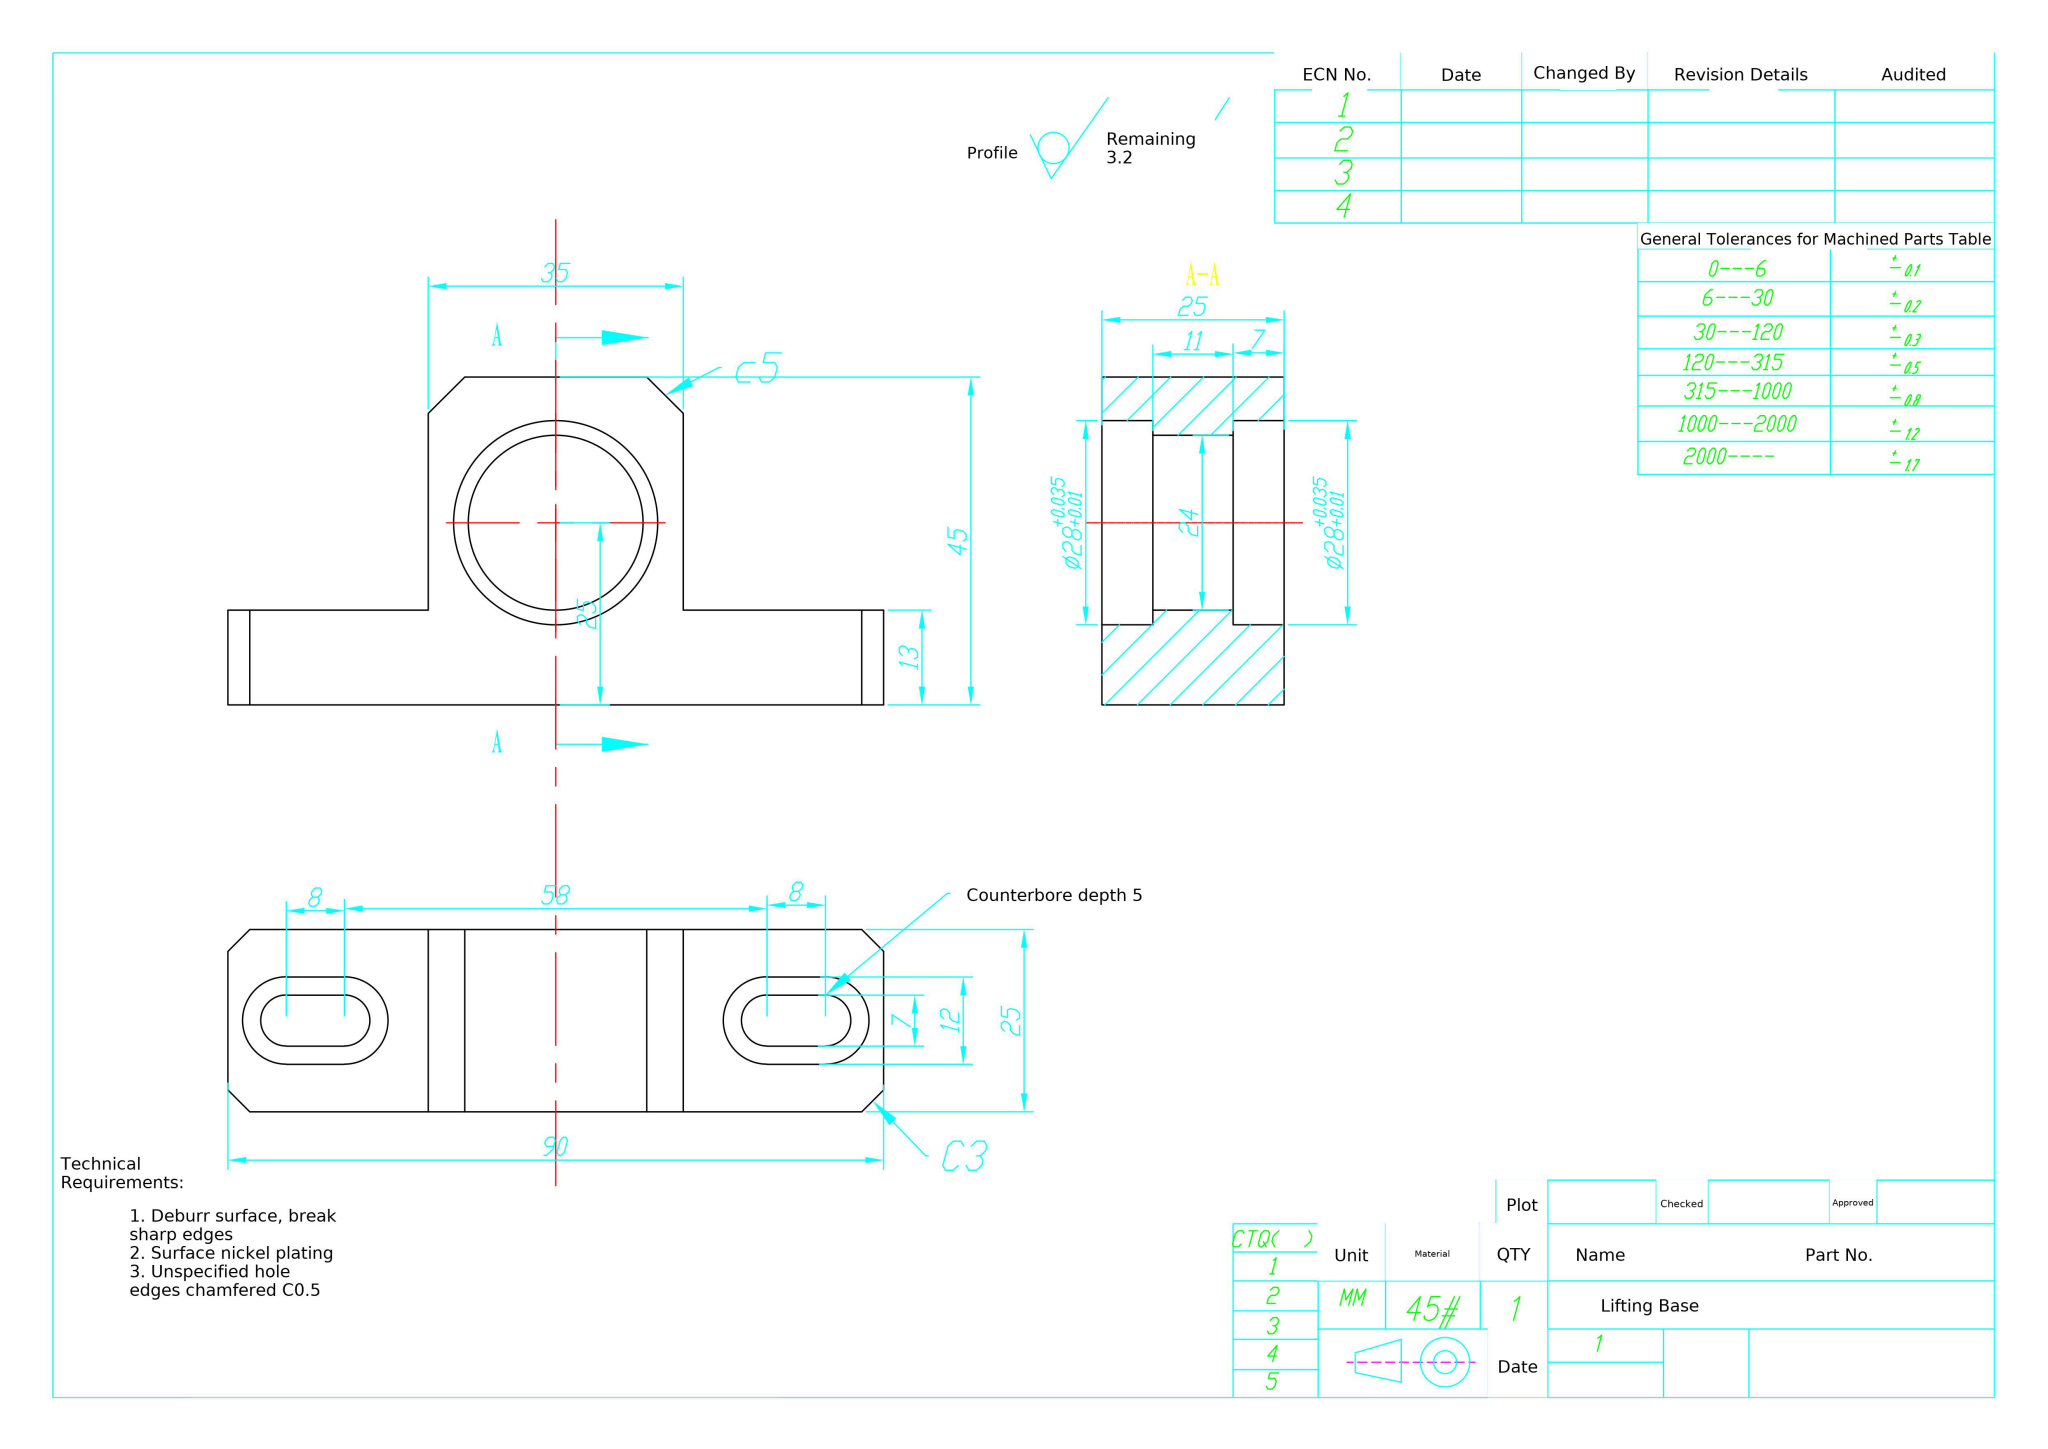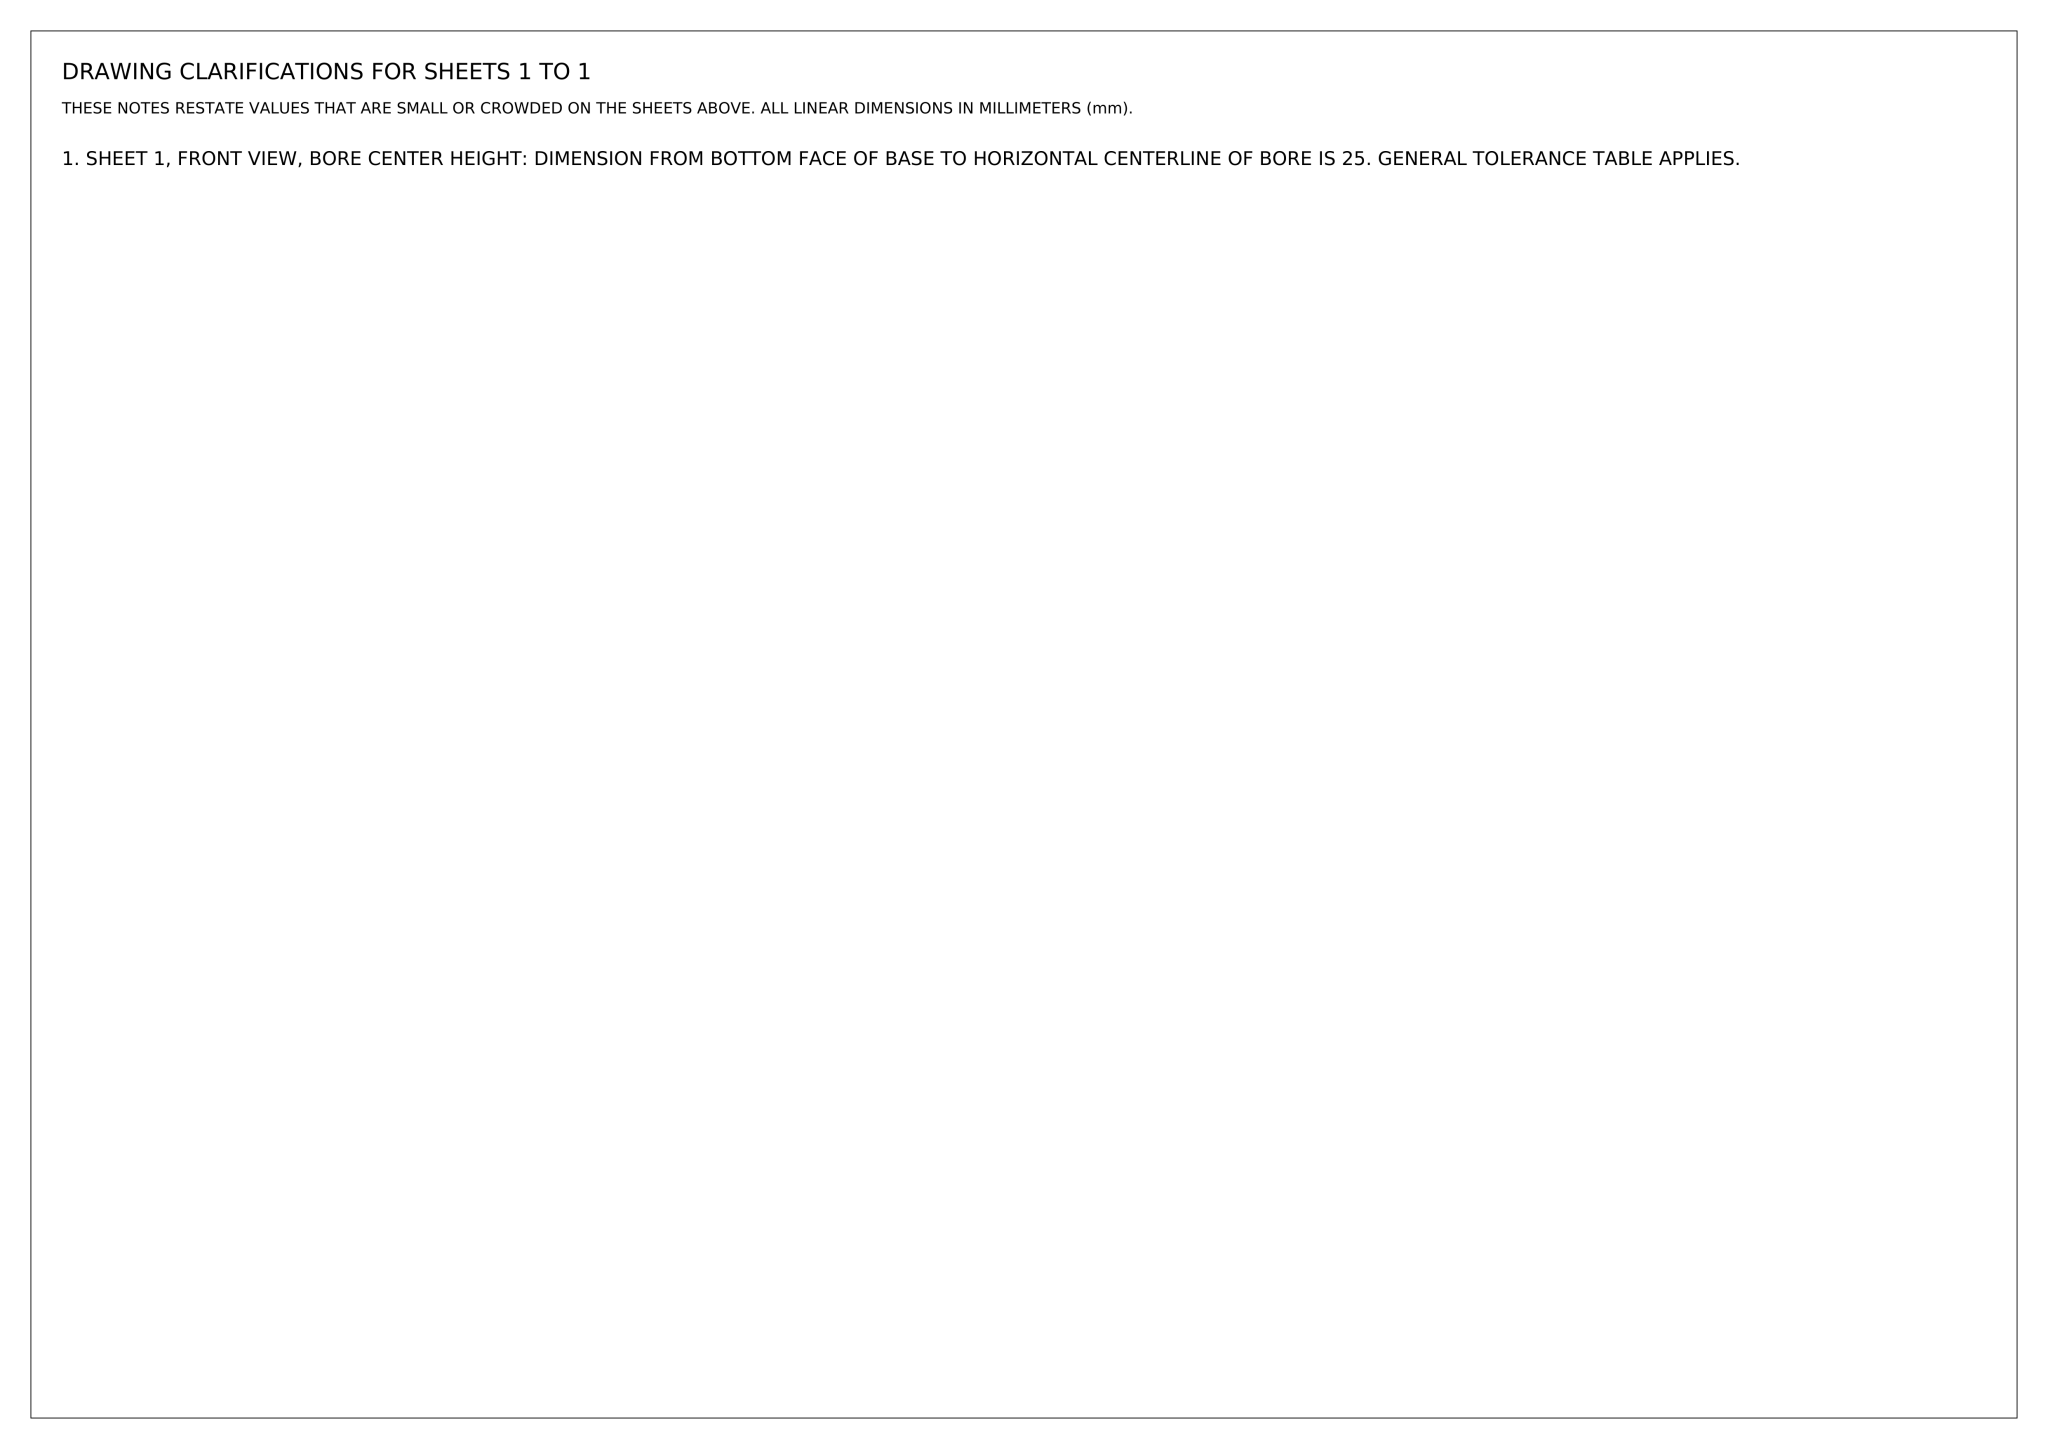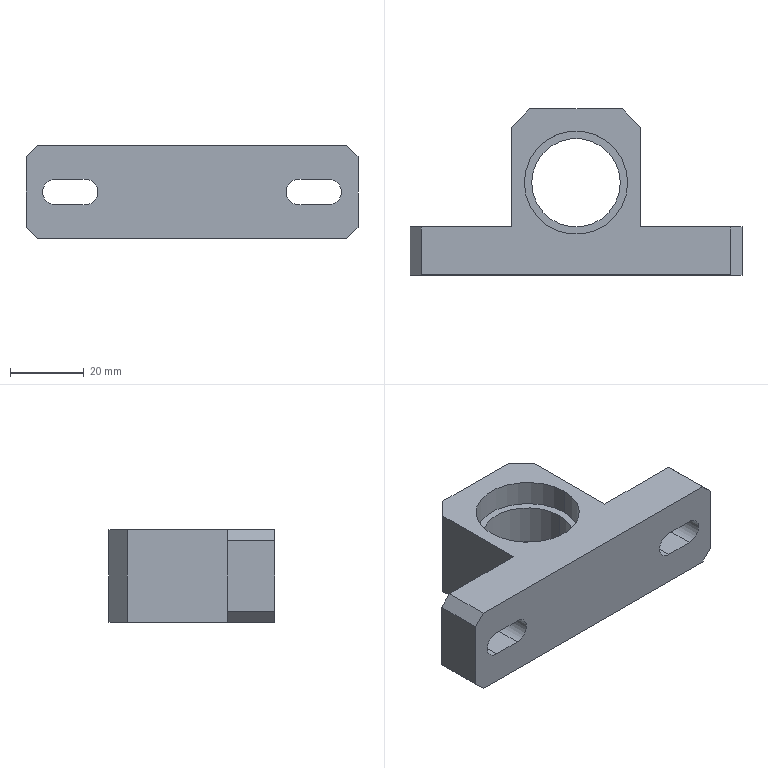Part | NX | mm | 1 solid | 42 faces | box 90 x 45 x 25 mm | volume 39191 mm3 | plane 28 | cylinder 14 | commonest cylinder face diameters 28 x4 7 x4 12 x4 24 x2